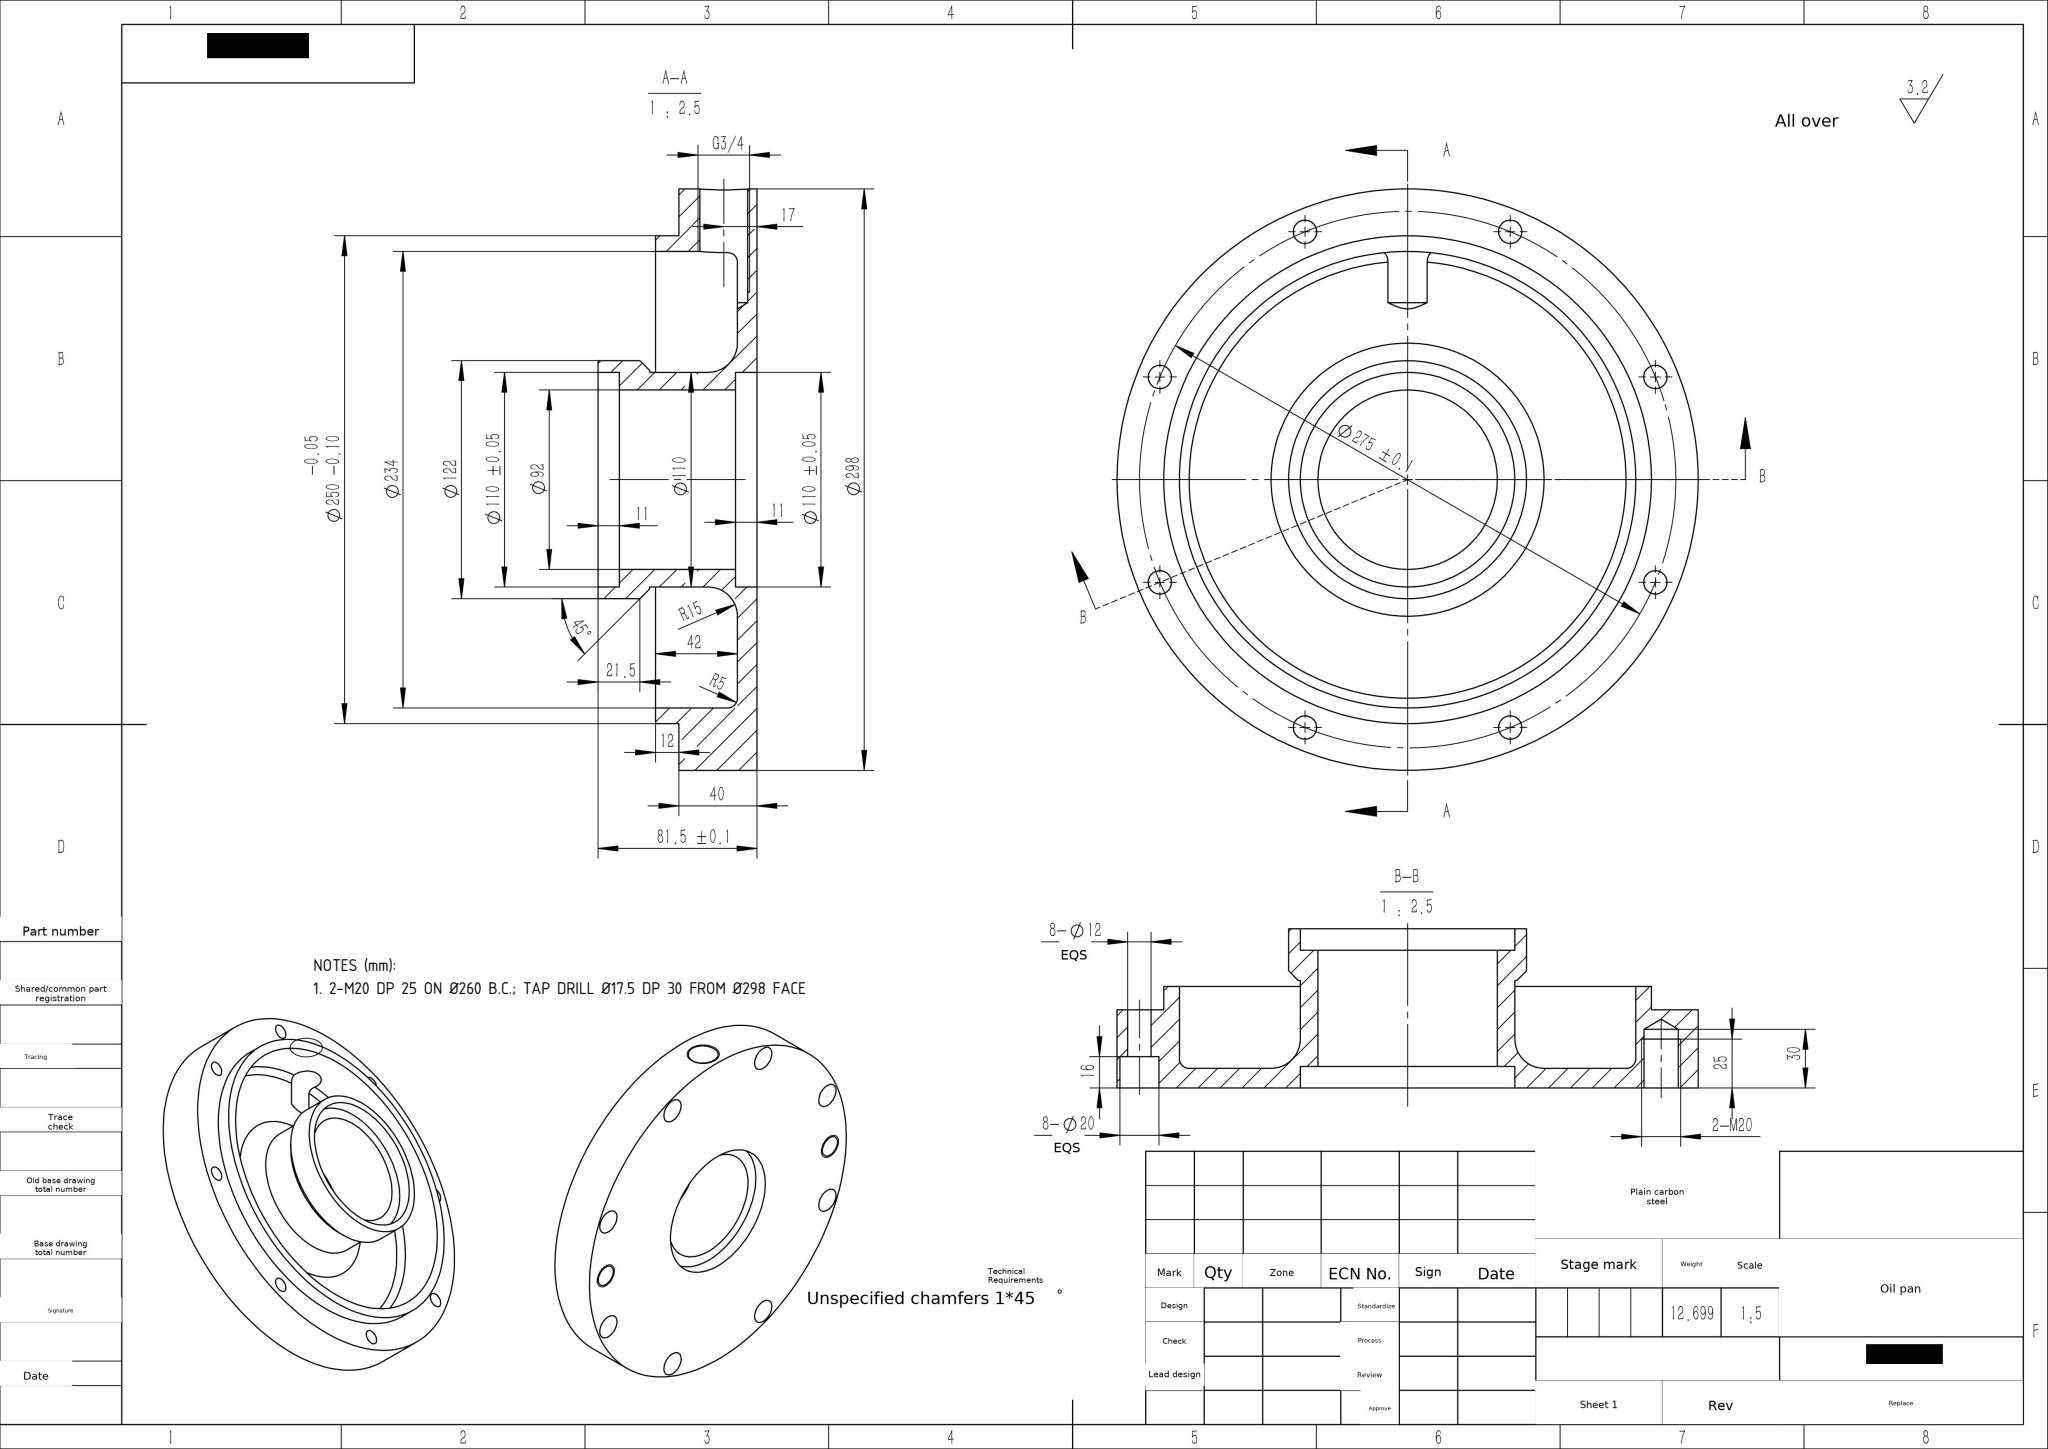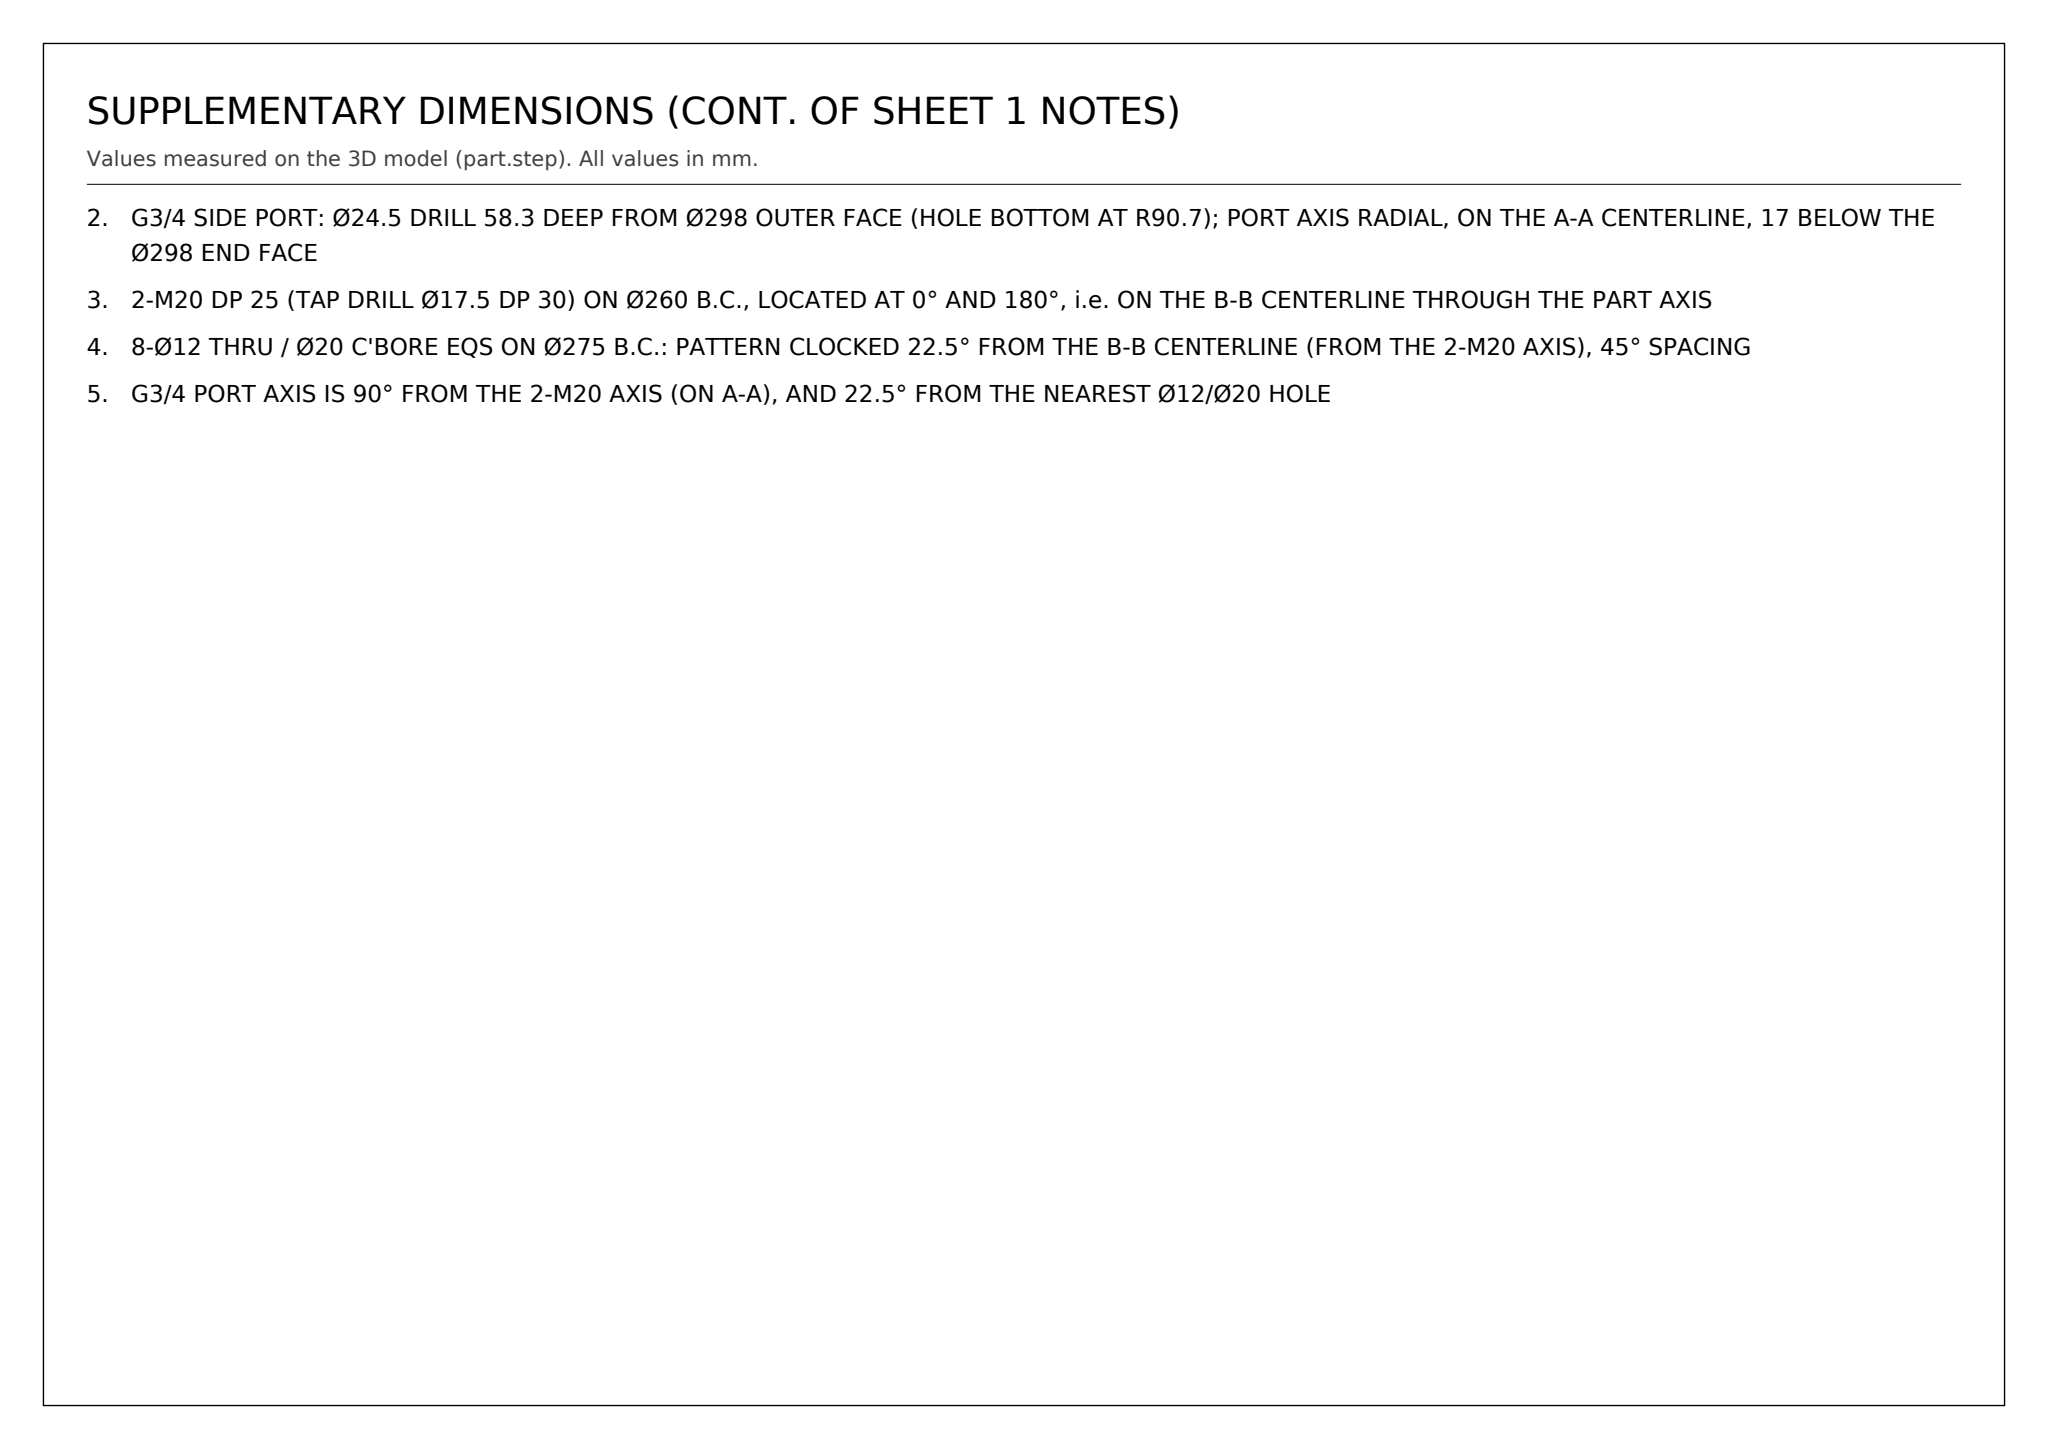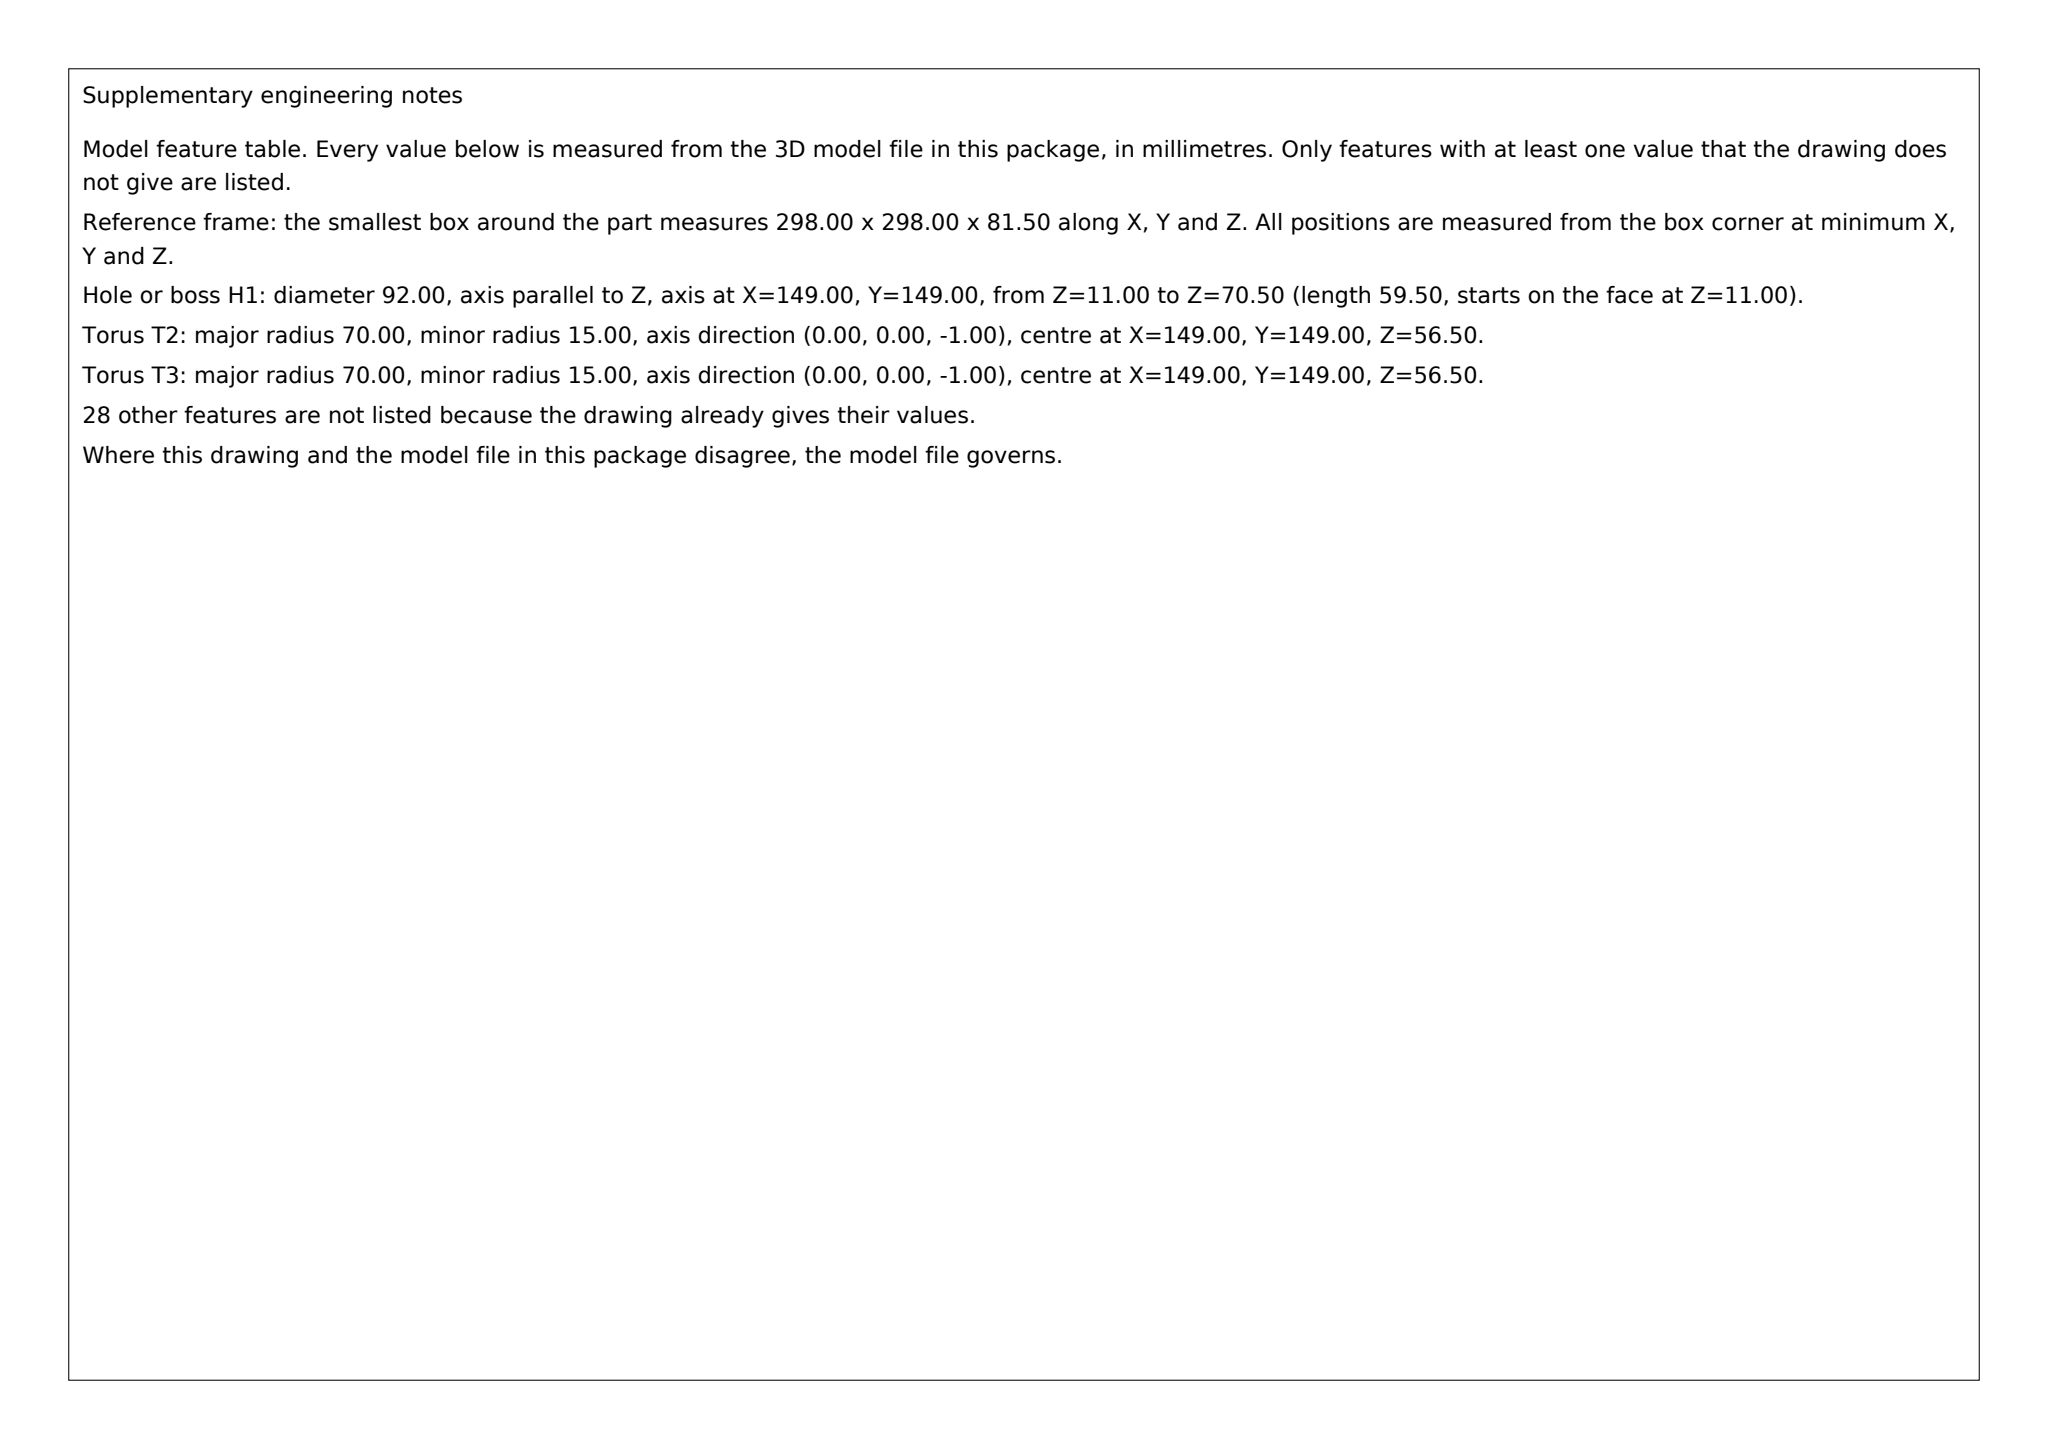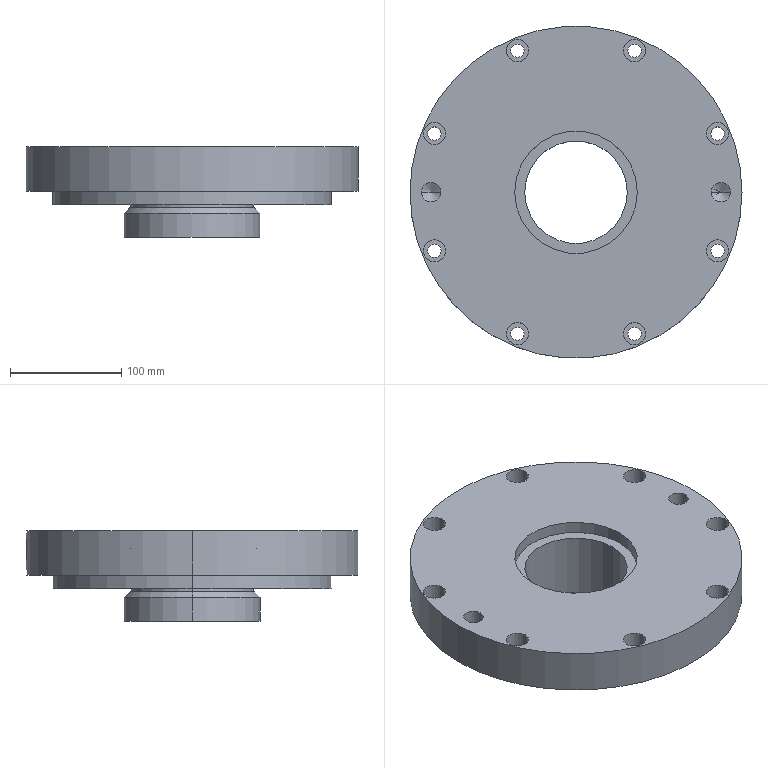Part | SolidWorks | mm | 1 solid | 83 faces | box 298 x 298 x 81.5 mm | volume 1627993 mm3 | cylinder 54 | plane 16 | cone 8 | torus 5 | commonest cylinder face diameters 20 x16 12 x16 110 x6 17.5 x4 24.5 x2 122 x2 234 x2 250 x2
Drawing notes:
2-M20 DP 25 ON Ø260 B.C.; TAP DRILL Ø17.5 DP 30 FROM Ø298 FACE | from the solid: Ø17.5 z-cyl L=30 at (19,149) & (279,149) = R130 (Ø260 BC) from Ø298 centre 149,149; 118° drill cone ref dia 17.5; boss hts 25/30 per z-planes 70.5/71.5/81.5
G3/4 SIDE PORT: Ø24.5 DRILL 58.3 DEEP FROM Ø298 OUTER FACE (HOLE BOTTOM AT R90.7); PORT AXIS RADIAL, ON THE A-A CENTERLINE, 17 BELOW THE Ø298 END FACE | from the solid: cylinders: hole/bore Ø24.5 axis y at [149.0, null, 64.5] from 239.7 to 298.0 (bbox z max 81.5, so axis 17 below top face); cone 118° ref dia 24.5 at drill point
2-M20 DP 25 (TAP DRILL Ø17.5 DP 30) ON Ø260 B.C., LOCATED AT 0° AND 180°, i.e. ON THE B-B CENTERLINE THROUGH THE PART AXIS | from the solid: cylinders: two Ø17.5 holes at [19.0,149.0] and [279.0,149.0], part axis at [149.0,149.0] → R130 (Ø260 B.C.) on the X axis
8-Ø12 THRU / Ø20 C'BORE EQS ON Ø275 B.C.: PATTERN CLOCKED 22.5° FROM THE B-B CENTERLINE (FROM THE 2-M20 AXIS), 45° SPACING | from the solid: cylinders: Ø12/Ø20 holes at [201.6,22.0], [276.0,96.4], etc.; from axis [149.0,149.0] gives R137.5 (Ø275) at 22.5°+n*45°
G3/4 PORT AXIS IS 90° FROM THE 2-M20 AXIS (ON A-A), AND 22.5° FROM THE NEAREST Ø12/Ø20 HOLE | from the solid: cylinders: Ø24.5 port axis at x=149.0, y to 298.0 (Y axis); Ø17.5 holes on X axis; Ø12 holes at 22.5°+n*45°
build123d program:
from build123d import *

# Parameters (mm, degrees)
SKETCH1_R               = 149
BOSS_EXTRUDE1_DEPTH     = 40
SKETCH2_R               = 125
SKETCH2_R_2             = 117
BOSS_EXTRUDE2_DEPTH     = 12
SKETCH3_R               = 61
BOSS_EXTRUDE3_DEPTH     = 41.5
SKETCH4_R               = 46
CUT_EXTRUDE1_DEPTH      = 226.93
SKETCH5_R               = 55
CUT_EXTRUDE2_DEPTH      = 11
CUT_EXTRUDE4_DEPTH      = 15
CUT_EXTRUDE4_DEPTH_BACK = 30
SKETCH7_R               = 117
SKETCH7_R_2             = 55
SKETCH9_R               = 6
CUT_EXTRUDE5_DEPTH      = 215.766
G3_4_TAPPED_HOLE1_D     = 24.5
G3_4_TAPPED_HOLE1_DEPTH = 58.32
G3_4_TAPPED_HOLE1_TIP   = 7.361
SKETCH11_R              = 10
CUT_EXTRUDE6_DEPTH      = 16
CIRPATTERN1_COUNT       = 8
FILLET1_R               = 15
FILLET2_R               = 5
CUT_EXTRUDE7_START      = -11
SKETCH6_R               = 55
CUT_EXTRUDE7_DEPTH      = 11
CHAMFER1_SIZE           = 5
CIRPATTERN2_COUNT       = 2


with BuildPart() as part:
    # Sketch1 → Boss-Extrude1 (new body)
    with BuildSketch(Plane.XY):
        Circle(SKETCH1_R)
    extrude(amount=BOSS_EXTRUDE1_DEPTH)

    # Sketch2 → Boss-Extrude2 (add)
    with BuildSketch(Plane(origin=(0, 0, 0), x_dir=(-1, 0, 0), z_dir=(0, 0, -1))):
        with Locations(Location((0, 0, 0), (0, 0, 180))):
            Circle(SKETCH2_R)
        Circle(SKETCH2_R_2, mode=Mode.SUBTRACT)
    extrude(amount=BOSS_EXTRUDE2_DEPTH)

    # Sketch3 → Boss-Extrude3 (add)
    with BuildSketch(Plane(origin=(0, 0, 0), x_dir=(-1, 0, 0), z_dir=(0, 0, -1))):
        with Locations(Location((0, 0, 0), (0, 0, 180))):
            Circle(SKETCH3_R)
    extrude(amount=BOSS_EXTRUDE3_DEPTH)

    # Sketch4 → Cut-Extrude1 (cut, through all)
    with BuildSketch(Plane.XY.offset(40)):
        Circle(SKETCH4_R)
    extrude(amount=-CUT_EXTRUDE1_DEPTH, mode=Mode.SUBTRACT)

    # Sketch5 → Cut-Extrude2 (cut)
    with BuildSketch(Plane(origin=(0, 0, -41.5), x_dir=(-1, 0, 0), z_dir=(0, 0, -1))):
        Circle(SKETCH5_R)
    extrude(amount=-CUT_EXTRUDE2_DEPTH, mode=Mode.SUBTRACT)

    # Sketch7 → Cut-Extrude4 (cut, two sides: drawn at the far end of the back side and taken through both)
    with BuildSketch(Plane(origin=(0, 0, 0), x_dir=(-1, 0, 0), z_dir=(0, 0, -1)).offset(-CUT_EXTRUDE4_DEPTH_BACK)):
        Circle(SKETCH7_R)
        Circle(SKETCH7_R_2, mode=Mode.SUBTRACT)
    extrude(amount=CUT_EXTRUDE4_DEPTH + CUT_EXTRUDE4_DEPTH_BACK, mode=Mode.SUBTRACT)

    # Sketch9 → Cut-Extrude5 (cut, through all)
    with BuildSketch(Plane(origin=(0, 0, 0), x_dir=(-1, 0, 0), z_dir=(0, 0, -1))):
        with Locations((-52.619, 127.033)):
            Circle(SKETCH9_R)
        with Locations((52.619, 127.033)):
            Circle(SKETCH9_R)
        with Locations((127.033, 52.619)):
            Circle(SKETCH9_R)
        with Locations((127.033, -52.619)):
            Circle(SKETCH9_R)
        with Locations((52.619, -127.033)):
            Circle(SKETCH9_R)
        with Locations((-52.619, -127.033)):
            Circle(SKETCH9_R)
        with Locations((-127.033, -52.619)):
            Circle(SKETCH9_R)
        with Locations((-127.033, 52.619)):
            Circle(SKETCH9_R)
    extrude(amount=-CUT_EXTRUDE5_DEPTH, mode=Mode.SUBTRACT)

    # G3_4 Tapped Hole1
    with Locations(Plane(origin=(0, 149, 23), x_dir=(1, 0, 0), z_dir=(0, 1, 0))):
        with Locations((0, 0)):
            Hole(G3_4_TAPPED_HOLE1_D / 2, depth=G3_4_TAPPED_HOLE1_DEPTH)
            with Locations((0, 0, -(G3_4_TAPPED_HOLE1_DEPTH + G3_4_TAPPED_HOLE1_TIP / 2))):  # 118° drill point
                Cone(0, G3_4_TAPPED_HOLE1_D / 2, G3_4_TAPPED_HOLE1_TIP, mode=Mode.SUBTRACT)

    # Sketch11 → Cut-Extrude6 (cut)
    with BuildSketch(Plane.XY.offset(40)):
        with Locations((-52.619, 127.033)):
            Circle(SKETCH11_R)
    cut_extrude6 = extrude(amount=-CUT_EXTRUDE6_DEPTH, mode=Mode.SUBTRACT)

    # CirPattern1: Cut-Extrude6 ×8 about axis
    cirpattern1_axis = Axis((0, 0, 0), (0, 0, 1))
    for i in range(1, CIRPATTERN1_COUNT):
        add(cut_extrude6.rotate(cirpattern1_axis, i * 360 / CIRPATTERN1_COUNT), mode=Mode.SUBTRACT)

    # Fillet1
    fillet1_edges = [part.edges().sort_by_distance(p)[0] for p in [
        (55, 0, 30),
    ]]
    fillet(fillet1_edges, radius=FILLET1_R)

    # Fillet2
    fillet2_edges = [part.edges().sort_by_distance(p)[0] for p in [
        (79.097, -86.213, 30),
    ]]
    fillet(fillet2_edges, radius=FILLET2_R)

    # Sketch6 → Cut-Extrude7 (cut)
    with BuildSketch(Plane.XY.offset(40).offset(CUT_EXTRUDE7_START)):
        with Locations(Location((0, 0, 0), (0, 0, 180))):
            Circle(SKETCH6_R)
    extrude(amount=CUT_EXTRUDE7_DEPTH, mode=Mode.SUBTRACT)

    # Chamfer1
    chamfer1_edges = [part.edges().sort_by_distance(p)[0] for p in [
        (-61, 0, -15),
    ]]
    chamfer(chamfer1_edges, length=CHAMFER1_SIZE)

    # Sketch14 → M20 Tapped Hole1 (revolve, cut)
    with BuildSketch(Plane(origin=(-130, 0, 40), x_dir=(0, -1, 0), z_dir=(1, 0, 0))):
        Polygon((0, 0), (0, 35.258), (8.75, 30), (8.75, 0), align=None)
    m20_tapped_hole1 = revolve(axis=Axis((-130, 0, 46.35), (0, 0, -1)), mode=Mode.SUBTRACT)

    # CirPattern2: M20 Tapped Hole1 ×2 about axis
    cirpattern2_axis = Axis((0, 0, 0), (0, 0, 1))
    for i in range(1, CIRPATTERN2_COUNT):
        add(m20_tapped_hole1.rotate(cirpattern2_axis, i * 360 / CIRPATTERN2_COUNT), mode=Mode.SUBTRACT)


solid = part.part